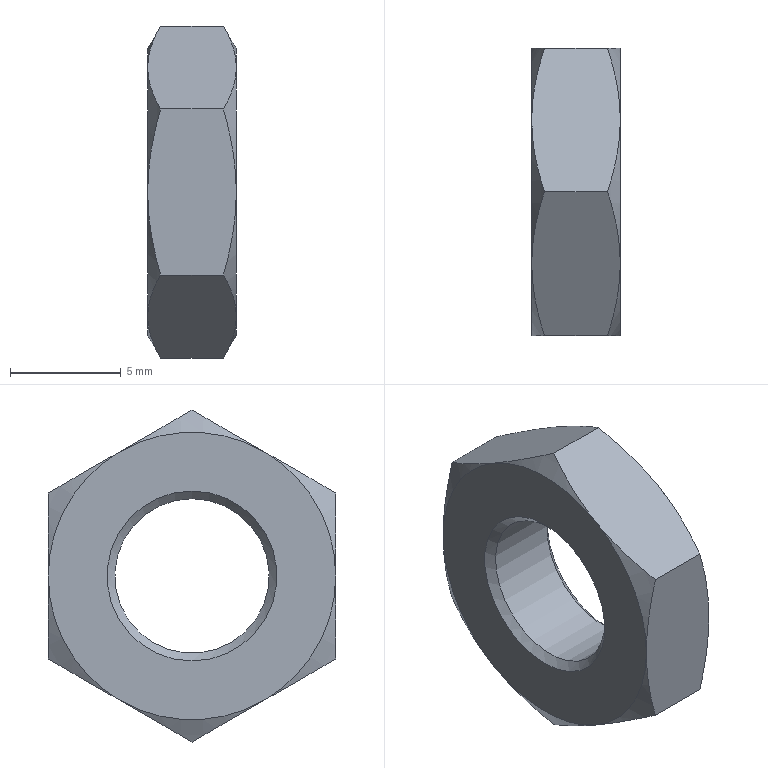Component | NX | GB-T6172_1-2000_M8X1_25 | 1 solid | 23 faces | volume 425 mm3 | cone 14 | plane 8 | cylinder 1 | commonest cylinder face diameters 6.985 x1